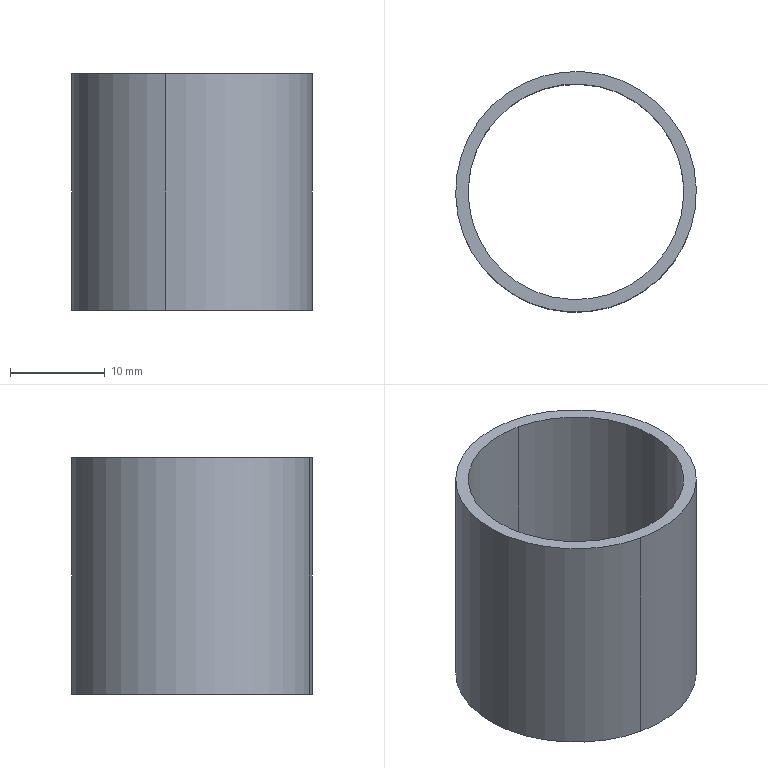Component | SolidWorks | TM-50LensCS-1 | 1 solid | 6 faces | box 25.4 x 25.4 x 25 mm | volume 2507 mm3 | cylinder 4 | plane 2 | commonest cylinder face diameters 22.748 x2 25.4 x2
build123d program:
from build123d import *

# Parameters (mm, degrees)
SKETCH1_R           = 12.7
SKETCH1_R_2         = 11.374
BOSS_EXTRUDE1_DEPTH = 25


with BuildPart() as part:
    # Sketch1 → Boss-Extrude1 (new body)
    with BuildSketch(Plane.XY):
        Circle(SKETCH1_R)
        Circle(SKETCH1_R_2, mode=Mode.SUBTRACT)
    extrude(amount=BOSS_EXTRUDE1_DEPTH)


solid = part.part

# Placed as in the assembly
solid = solid.moved(Location((-146.071, 219.819, 387.399), (0, 0, 0)))
STEP:
#1=COLOUR_RGB('',0.7922,0.8196,0.9333);
#2=FILL_AREA_STYLE_COLOUR('',#1);
#3=FILL_AREA_STYLE('',(#2));
#4=SURFACE_STYLE_FILL_AREA(#3);
#5=SURFACE_SIDE_STYLE('',(#4));
#6=SURFACE_STYLE_USAGE(.BOTH.,#5);
#7=PRESENTATION_STYLE_ASSIGNMENT((#6));
#8=CARTESIAN_POINT('',(-5.654,9.092,16.236));
#9=VERTEX_POINT('',#8);
#10=CARTESIAN_POINT('',(-5.848,8.217,16.236));
#11=VERTEX_POINT('',#10);
#12=CARTESIAN_POINT('',(-5.751,8.654,16.236));
#13=DIRECTION('',(0.,-0.,1.));
#14=DIRECTION('',(-0.2161,-0.9764,0.));
#15=AXIS2_PLACEMENT_3D('',#12,#13,#14);
#16=CIRCLE('',#15,0.4478);
#17=EDGE_CURVE('',#9,#11,#16,.T.);
#18=ORIENTED_EDGE('',*,*,#17,.T.);
#19=CARTESIAN_POINT('',(-5.848,8.217,15.252));
#20=VERTEX_POINT('',#19);
#21=CARTESIAN_POINT('',(-5.848,8.217,16.236));
#22=DIRECTION('',(-0.,0.,-1.));
#23=VECTOR('',#22,39.37);
#24=LINE('',#21,#23);
#25=EDGE_CURVE('',#11,#20,#24,.T.);
#26=ORIENTED_EDGE('',*,*,#25,.T.);
#27=CARTESIAN_POINT('',(-5.654,9.092,15.252));
#28=VERTEX_POINT('',#27);
#29=CARTESIAN_POINT('',(-5.751,8.654,15.252));
#30=DIRECTION('',(0.,-0.,1.));
#31=DIRECTION('',(-0.2161,-0.9764,0.));
#32=AXIS2_PLACEMENT_3D('',#29,#30,#31);
#33=CIRCLE('',#32,0.4478);
#34=EDGE_CURVE('',#28,#20,#33,.T.);
#35=ORIENTED_EDGE('',*,*,#34,.F.);
#36=CARTESIAN_POINT('',(-5.654,9.092,16.236));
#37=DIRECTION('',(-0.,0.,-1.));
#38=VECTOR('',#37,39.37);
#39=LINE('',#36,#38);
#40=EDGE_CURVE('',#9,#28,#39,.T.);
#41=ORIENTED_EDGE('',*,*,#40,.F.);
#42=EDGE_LOOP('',(#18,#26,#35,#41));
#43=FACE_OUTER_BOUND('',#42,.T.);
#44=CARTESIAN_POINT('',(-5.751,8.654,16.236));
#45=DIRECTION('',(-0.,0.,-1.));
#46=DIRECTION('',(0.2161,0.9764,0.));
#47=AXIS2_PLACEMENT_3D('',#44,#45,#46);
#48=CYLINDRICAL_SURFACE('',#47,0.4478);
#49=ADVANCED_FACE('',(#43),#48,.F.);
#50=CARTESIAN_POINT('',(-5.859,8.166,16.236));
#51=VERTEX_POINT('',#50);
#52=CARTESIAN_POINT('',(-5.643,9.142,16.236));
#53=VERTEX_POINT('',#52);
#54=CARTESIAN_POINT('',(-5.751,8.654,16.236));
#55=DIRECTION('',(0.,-0.,1.));
#56=DIRECTION('',(-0.2161,-0.9764,0.));
#57=AXIS2_PLACEMENT_3D('',#54,#55,#56);
#58=CIRCLE('',#57,0.5);
#59=EDGE_CURVE('',#51,#53,#58,.T.);
#60=ORIENTED_EDGE('',*,*,#59,.F.);
#61=CARTESIAN_POINT('',(-5.859,8.166,15.252));
#62=VERTEX_POINT('',#61);
#63=CARTESIAN_POINT('',(-5.859,8.166,16.236));
#64=DIRECTION('',(-0.,0.,-1.));
#65=VECTOR('',#64,39.37);
#66=LINE('',#63,#65);
#67=EDGE_CURVE('',#51,#62,#66,.T.);
#68=ORIENTED_EDGE('',*,*,#67,.T.);
#69=CARTESIAN_POINT('',(-5.643,9.142,15.252));
#70=VERTEX_POINT('',#69);
#71=CARTESIAN_POINT('',(-5.751,8.654,15.252));
#72=DIRECTION('',(0.,-0.,1.));
#73=DIRECTION('',(-0.2161,-0.9764,0.));
#74=AXIS2_PLACEMENT_3D('',#71,#72,#73);
#75=CIRCLE('',#74,0.5);
#76=EDGE_CURVE('',#62,#70,#75,.T.);
#77=ORIENTED_EDGE('',*,*,#76,.T.);
#78=CARTESIAN_POINT('',(-5.643,9.142,16.236));
#79=DIRECTION('',(-0.,0.,-1.));
#80=VECTOR('',#79,39.37);
#81=LINE('',#78,#80);
#82=EDGE_CURVE('',#53,#70,#81,.T.);
#83=ORIENTED_EDGE('',*,*,#82,.F.);
#84=EDGE_LOOP('',(#60,#68,#77,#83));
#85=FACE_OUTER_BOUND('',#84,.T.);
#86=CARTESIAN_POINT('',(-5.751,8.654,16.236));
#87=DIRECTION('',(-0.,0.,-1.));
#88=DIRECTION('',(0.2161,0.9764,0.));
#89=AXIS2_PLACEMENT_3D('',#86,#87,#88);
#90=CYLINDRICAL_SURFACE('',#89,0.5);
#91=ADVANCED_FACE('',(#85),#90,.T.);
#92=CARTESIAN_POINT('',(-5.751,8.654,16.236));
#93=DIRECTION('',(0.,-0.,1.));
#94=DIRECTION('',(-0.2161,-0.9764,0.));
#95=AXIS2_PLACEMENT_3D('',#92,#93,#94);
#96=CIRCLE('',#95,0.5);
#97=EDGE_CURVE('',#53,#51,#96,.T.);
#98=ORIENTED_EDGE('',*,*,#97,.T.);
#99=ORIENTED_EDGE('',*,*,#59,.T.);
#100=EDGE_LOOP('',(#98,#99));
#101=FACE_OUTER_BOUND('',#100,.T.);
#102=ORIENTED_EDGE('',*,*,#17,.F.);
#103=CARTESIAN_POINT('',(-5.751,8.654,16.236));
#104=DIRECTION('',(0.,-0.,1.));
#105=DIRECTION('',(-0.2161,-0.9764,0.));
#106=AXIS2_PLACEMENT_3D('',#103,#104,#105);
#107=CIRCLE('',#106,0.4478);
#108=EDGE_CURVE('',#11,#9,#107,.T.);
#109=ORIENTED_EDGE('',*,*,#108,.F.);
#110=EDGE_LOOP('',(#102,#109));
#111=FACE_BOUND('',#110,.T.);
#112=CARTESIAN_POINT('',(-5.751,8.654,16.236));
#113=DIRECTION('',(0.,-0.,1.));
#114=DIRECTION('',(-0.2161,-0.9764,0.));
#115=AXIS2_PLACEMENT_3D('',#112,#113,#114);
#116=PLANE('',#115);
#117=ADVANCED_FACE('',(#101,#111),#116,.T.);
#118=CARTESIAN_POINT('',(-5.751,8.654,15.252));
#119=DIRECTION('',(0.,-0.,1.));
#120=DIRECTION('',(-0.2161,-0.9764,0.));
#121=AXIS2_PLACEMENT_3D('',#118,#119,#120);
#122=CIRCLE('',#121,0.5);
#123=EDGE_CURVE('',#70,#62,#122,.T.);
#124=ORIENTED_EDGE('',*,*,#123,.F.);
#125=ORIENTED_EDGE('',*,*,#76,.F.);
#126=EDGE_LOOP('',(#124,#125));
#127=FACE_OUTER_BOUND('',#126,.T.);
#128=ORIENTED_EDGE('',*,*,#34,.T.);
#129=CARTESIAN_POINT('',(-5.751,8.654,15.252));
#130=DIRECTION('',(0.,-0.,1.));
#131=DIRECTION('',(-0.2161,-0.9764,0.));
#132=AXIS2_PLACEMENT_3D('',#129,#130,#131);
#133=CIRCLE('',#132,0.4478);
#134=EDGE_CURVE('',#20,#28,#133,.T.);
#135=ORIENTED_EDGE('',*,*,#134,.T.);
#136=EDGE_LOOP('',(#128,#135));
#137=FACE_BOUND('',#136,.T.);
#138=CARTESIAN_POINT('',(-5.751,8.654,15.252));
#139=DIRECTION('',(0.,-0.,1.));
#140=DIRECTION('',(-0.2161,-0.9764,0.));
#141=AXIS2_PLACEMENT_3D('',#138,#139,#140);
#142=PLANE('',#141);
#143=ADVANCED_FACE('',(#127,#137),#142,.F.);
#144=ORIENTED_EDGE('',*,*,#67,.F.);
#145=ORIENTED_EDGE('',*,*,#97,.F.);
#146=ORIENTED_EDGE('',*,*,#82,.T.);
#147=ORIENTED_EDGE('',*,*,#123,.T.);
#148=EDGE_LOOP('',(#144,#145,#146,#147));
#149=FACE_OUTER_BOUND('',#148,.T.);
#150=CARTESIAN_POINT('',(-5.751,8.654,16.236));
#151=DIRECTION('',(-0.,0.,-1.));
#152=DIRECTION('',(0.2161,0.9764,0.));
#153=AXIS2_PLACEMENT_3D('',#150,#151,#152);
#154=CYLINDRICAL_SURFACE('',#153,0.5);
#155=ADVANCED_FACE('',(#149),#154,.T.);
#156=ORIENTED_EDGE('',*,*,#25,.F.);
#157=ORIENTED_EDGE('',*,*,#108,.T.);
#158=ORIENTED_EDGE('',*,*,#40,.T.);
#159=ORIENTED_EDGE('',*,*,#134,.F.);
#160=EDGE_LOOP('',(#156,#157,#158,#159));
#161=FACE_OUTER_BOUND('',#160,.T.);
#162=CARTESIAN_POINT('',(-5.751,8.654,16.236));
#163=DIRECTION('',(-0.,0.,-1.));
#164=DIRECTION('',(0.2161,0.9764,0.));
#165=AXIS2_PLACEMENT_3D('',#162,#163,#164);
#166=CYLINDRICAL_SURFACE('',#165,0.4478);
#167=ADVANCED_FACE('',(#161),#166,.F.);
#168=CLOSED_SHELL('',(#49,#91,#117,#143,#155,#167));
#169=MANIFOLD_SOLID_BREP('',#168);
#170=STYLED_ITEM('',(#7),#169);
#171=(LENGTH_UNIT()NAMED_UNIT(*)SI_UNIT($,.METRE.));
#172=LENGTH_MEASURE_WITH_UNIT(LENGTH_MEASURE(0.0254),#171);
#173=DIMENSIONAL_EXPONENTS(1.,0.,0.,0.,0.,0.,0.);
#174=(CONVERSION_BASED_UNIT('',#172)LENGTH_UNIT()NAMED_UNIT(#173));
#175=UNCERTAINTY_MEASURE_WITH_UNIT(LENGTH_MEASURE(0.00001),#174,'','');
#176=(NAMED_UNIT(*)PLANE_ANGLE_UNIT()SI_UNIT($,.RADIAN.));
#177=(NAMED_UNIT(*)SI_UNIT($,.STERADIAN.)SOLID_ANGLE_UNIT());
#178=(GEOMETRIC_REPRESENTATION_CONTEXT(3)GLOBAL_UNCERTAINTY_ASSIGNED_CONTEXT((#175))GLOBAL_UNIT_ASSIGNED_CONTEXT((#174,#176,#177))REPRESENTATION_CONTEXT('',''));
#179=MECHANICAL_DESIGN_GEOMETRIC_PRESENTATION_REPRESENTATION('',(#170),#178);
#180=PRESENTATION_LAYER_ASSIGNMENT('','',(#170));
#181=CARTESIAN_POINT('',(0.,0.,0.));
#182=DIRECTION('',(0.,0.,1.));
#183=DIRECTION('',(1.,0.,0.));
#184=AXIS2_PLACEMENT_3D('',#181,#182,#183);
#185=(LENGTH_UNIT()NAMED_UNIT(*)SI_UNIT($,.METRE.));
#186=LENGTH_MEASURE_WITH_UNIT(LENGTH_MEASURE(0.0254),#185);
#187=DIMENSIONAL_EXPONENTS(1.,0.,0.,0.,0.,0.,0.);
#188=(CONVERSION_BASED_UNIT('',#186)LENGTH_UNIT()NAMED_UNIT(#187));
#189=UNCERTAINTY_MEASURE_WITH_UNIT(LENGTH_MEASURE(0.00001),#188,'','');
#190=(NAMED_UNIT(*)PLANE_ANGLE_UNIT()SI_UNIT($,.RADIAN.));
#191=(NAMED_UNIT(*)SI_UNIT($,.STERADIAN.)SOLID_ANGLE_UNIT());
#192=(GEOMETRIC_REPRESENTATION_CONTEXT(3)GLOBAL_UNCERTAINTY_ASSIGNED_CONTEXT((#189))GLOBAL_UNIT_ASSIGNED_CONTEXT((#188,#190,#191))REPRESENTATION_CONTEXT('',''));
#193=ADVANCED_BREP_SHAPE_REPRESENTATION('',(#169,#184),#192);